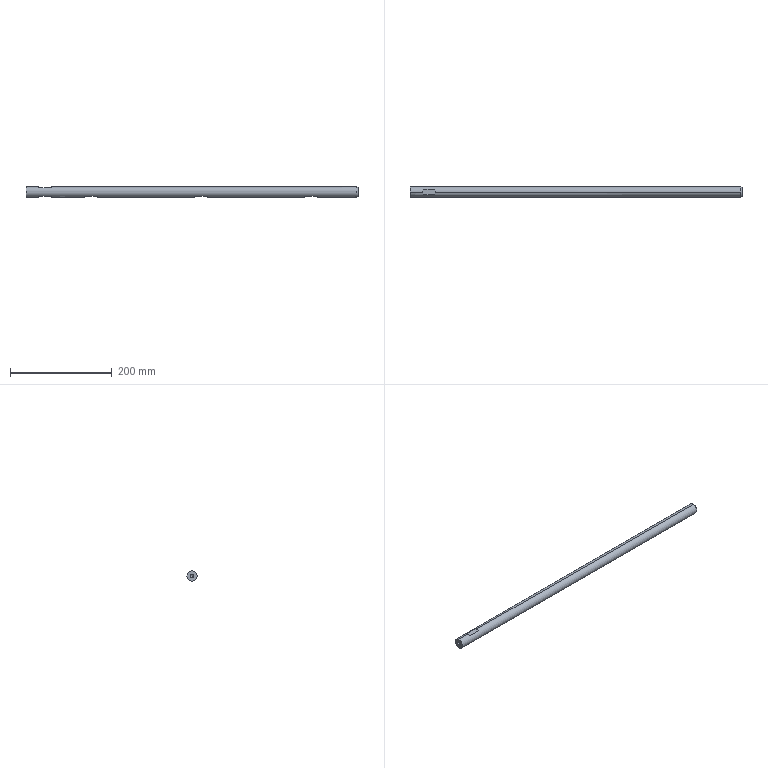CAM job | Mastercam | mm | 7 operations | part box 652 x 20 x 20
1. Contour (Ramp) | 4 - 10 平铣刀
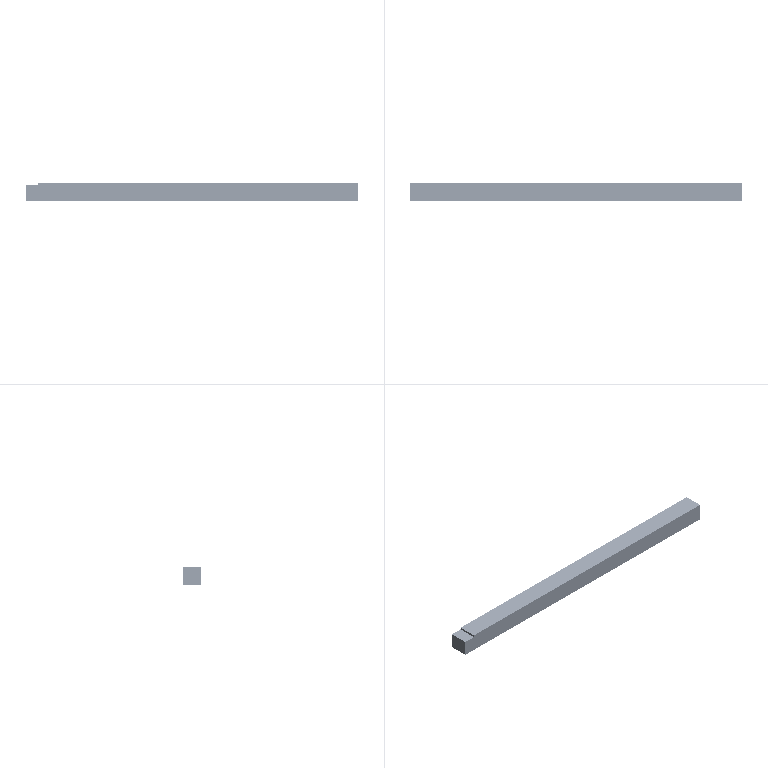2. Contour (2D) | 5 - 10 平铣刀
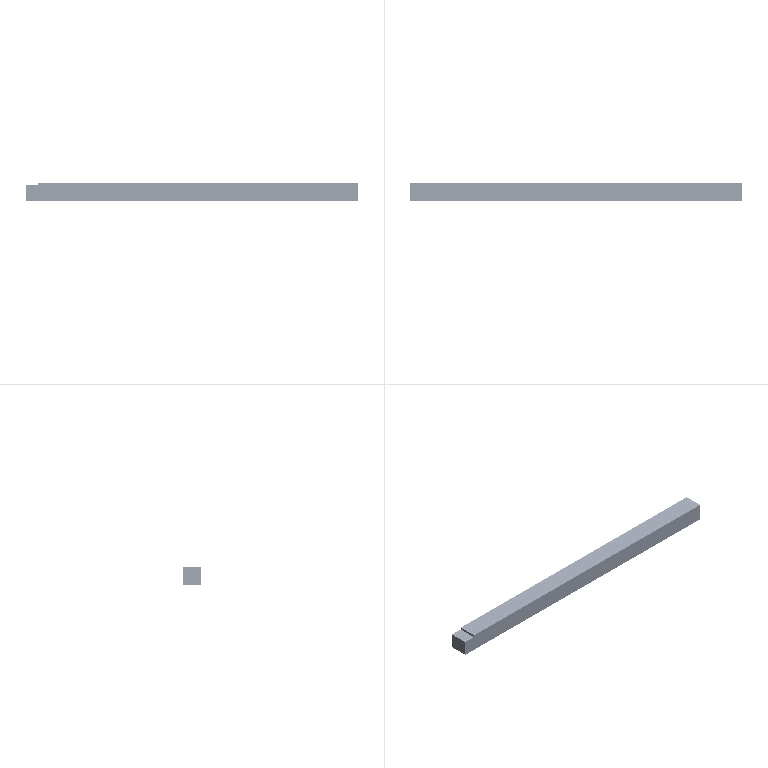3. Contour (Ramp) | 4 - 10 平铣刀
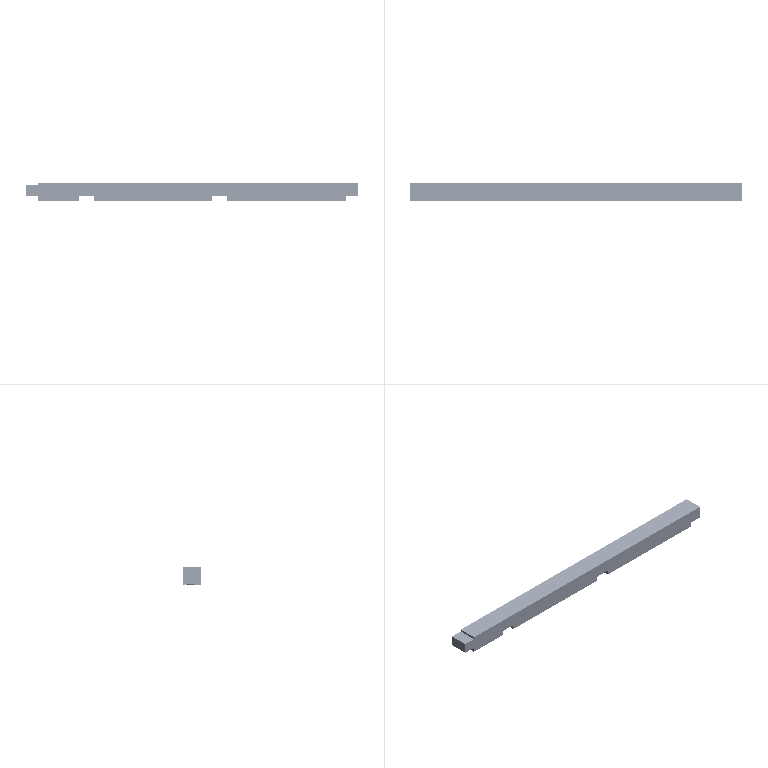4. Contour (2D) | 5 - 10 平铣刀
5. Drill/Counterbore | 3 - 4 倒角刀
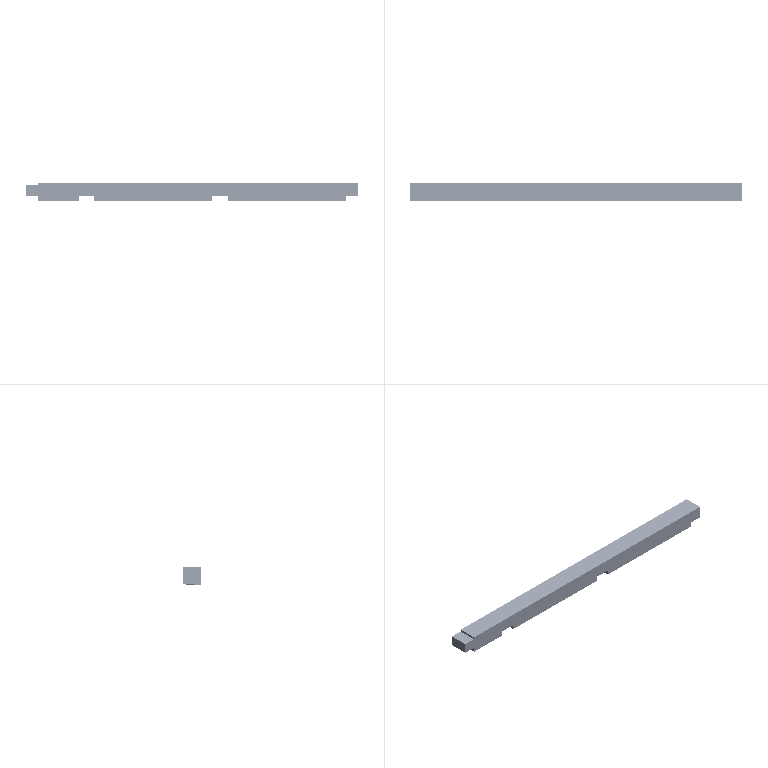6. Peck Drill | 6 - 3.3 钻头
7. Chamfer Drill | 3 - 4 倒角刀